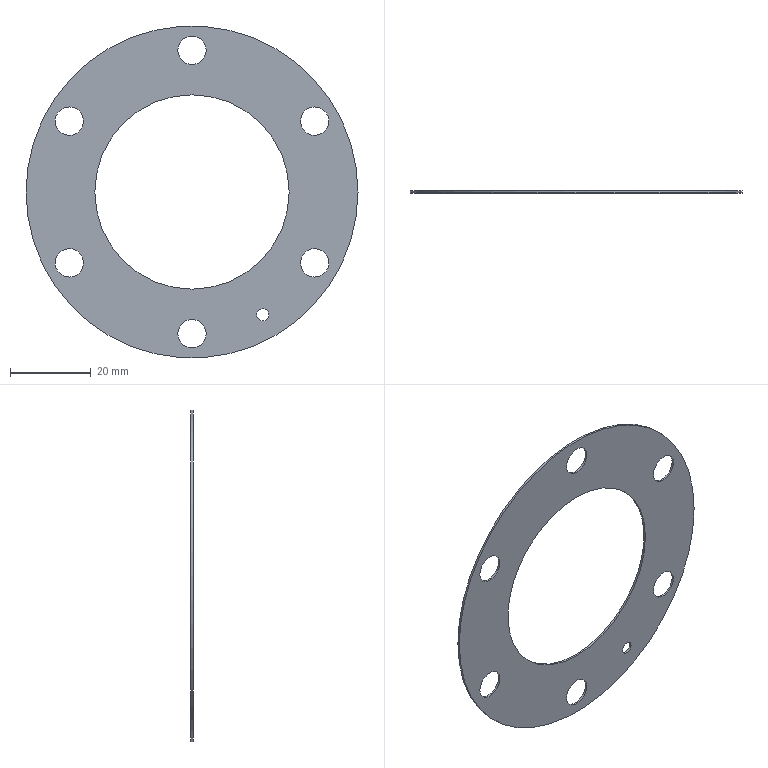Component | NX | GASKET | 1 solid | 11 faces | box 82 x 0.5 x 82 mm | volume 1617 mm3 | cylinder 9 | plane 2 | commonest cylinder face diameters 7 x6 3 x1 48 x1 82 x1
STEP:
#1=CARTESIAN_POINT('',(0.,0.,0.));
#2=DIRECTION('',(0.,0.,1.));
#3=DIRECTION('',(1.,0.,0.));
#4=AXIS2_PLACEMENT_3D('',#1,#2,#3);
#5=CARTESIAN_POINT('',(19.,-34.5,-25.811));
#6=VERTEX_POINT('',#5);
#7=CARTESIAN_POINT('',(17.5,-34.5,-25.811));
#8=DIRECTION('',(0.,1.,0.));
#9=DIRECTION('',(1.,0.,0.));
#10=AXIS2_PLACEMENT_3D('',#7,#8,#9);
#11=CIRCLE('',#10,1.5);
#12=CARTESIAN_POINT('',(17.5,-34.5,-25.811));
#13=DIRECTION('',(0.,1.,0.));
#14=DIRECTION('',(-1.,0.,0.));
#15=AXIS2_PLACEMENT_3D('',#12,#13,#14);
#16=CYLINDRICAL_SURFACE('',#15,1.5);
#17=CARTESIAN_POINT('',(3.142,0.));
#18=DIRECTION('',(1.,0.));
#19=VECTOR('',#18,1.);
#20=LINE('',#17,#19);
#21=(GEOMETRIC_REPRESENTATION_CONTEXT(2)PARAMETRIC_REPRESENTATION_CONTEXT()REPRESENTATION_CONTEXT('',''));
#22=DEFINITIONAL_REPRESENTATION('',(#20),#21);
#23=PCURVE('',#16,#22);
#24=CARTESIAN_POINT('',(15.155,-34.5,-4.25));
#25=DIRECTION('',(0.,1.,0.));
#26=DIRECTION('',(-1.,0.,0.));
#27=AXIS2_PLACEMENT_3D('',#24,#25,#26);
#28=PLANE('',#27);
#29=CARTESIAN_POINT('',(-2.345,-21.561));
#30=DIRECTION('',(-1.,0.));
#31=AXIS2_PLACEMENT_2D('',#29,#30);
#32=CIRCLE('',#31,1.5);
#33=(GEOMETRIC_REPRESENTATION_CONTEXT(2)PARAMETRIC_REPRESENTATION_CONTEXT()REPRESENTATION_CONTEXT('',''));
#34=DEFINITIONAL_REPRESENTATION('',(#32),#33);
#35=PCURVE('',#28,#34);
#36=SURFACE_CURVE('',#11,(#23,#35),.PCURVE_S1.);
#37=EDGE_CURVE('',#6,#6,#36,.T.);
#38=ORIENTED_EDGE('',*,*,#37,.T.);
#39=CARTESIAN_POINT('',(19.,-34.,-25.811));
#40=VERTEX_POINT('',#39);
#41=CARTESIAN_POINT('',(19.,-34.5,-25.811));
#42=CARTESIAN_POINT('',(19.,-34.,-25.811));
#43=B_SPLINE_CURVE_WITH_KNOTS('',1,(#41,#42),.UNSPECIFIED.,.F.,.F.,(2,2),(0.,0.5),.PIECEWISE_BEZIER_KNOTS.);
#44=CARTESIAN_POINT('',(9.425,0.));
#45=DIRECTION('',(0.,1.));
#46=VECTOR('',#45,1.);
#47=LINE('',#44,#46);
#48=(GEOMETRIC_REPRESENTATION_CONTEXT(2)PARAMETRIC_REPRESENTATION_CONTEXT()REPRESENTATION_CONTEXT('',''));
#49=DEFINITIONAL_REPRESENTATION('',(#47),#48);
#50=PCURVE('',#16,#49);
#51=CARTESIAN_POINT('',(3.142,0.));
#52=DIRECTION('',(0.,1.));
#53=VECTOR('',#52,1.);
#54=LINE('',#51,#53);
#55=(GEOMETRIC_REPRESENTATION_CONTEXT(2)PARAMETRIC_REPRESENTATION_CONTEXT()REPRESENTATION_CONTEXT('',''));
#56=DEFINITIONAL_REPRESENTATION('',(#54),#55);
#57=PCURVE('',#16,#56);
#58=SEAM_CURVE('',#43,(#50,#57),.PCURVE_S1.);
#59=EDGE_CURVE('',#6,#40,#58,.T.);
#60=ORIENTED_EDGE('',*,*,#59,.T.);
#61=CARTESIAN_POINT('',(17.5,-34.,-25.811));
#62=DIRECTION('',(0.,1.,0.));
#63=DIRECTION('',(1.,0.,0.));
#64=AXIS2_PLACEMENT_3D('',#61,#62,#63);
#65=CIRCLE('',#64,1.5);
#66=CARTESIAN_POINT('',(3.142,0.5));
#67=DIRECTION('',(1.,0.));
#68=VECTOR('',#67,1.);
#69=LINE('',#66,#68);
#70=(GEOMETRIC_REPRESENTATION_CONTEXT(2)PARAMETRIC_REPRESENTATION_CONTEXT()REPRESENTATION_CONTEXT('',''));
#71=DEFINITIONAL_REPRESENTATION('',(#69),#70);
#72=PCURVE('',#16,#71);
#73=CARTESIAN_POINT('',(15.155,-34.,-4.25));
#74=DIRECTION('',(0.,1.,0.));
#75=DIRECTION('',(-1.,0.,0.));
#76=AXIS2_PLACEMENT_3D('',#73,#74,#75);
#77=PLANE('',#76);
#78=CARTESIAN_POINT('',(-2.345,-21.561));
#79=DIRECTION('',(-1.,0.));
#80=AXIS2_PLACEMENT_2D('',#78,#79);
#81=CIRCLE('',#80,1.5);
#82=(GEOMETRIC_REPRESENTATION_CONTEXT(2)PARAMETRIC_REPRESENTATION_CONTEXT()REPRESENTATION_CONTEXT('',''));
#83=DEFINITIONAL_REPRESENTATION('',(#81),#82);
#84=PCURVE('',#77,#83);
#85=SURFACE_CURVE('',#65,(#72,#84),.PCURVE_S1.);
#86=EDGE_CURVE('',#40,#40,#85,.T.);
#87=ORIENTED_EDGE('',*,*,#86,.F.);
#88=ORIENTED_EDGE('',*,*,#59,.F.);
#89=EDGE_LOOP('',(#38,#60,#87,#88));
#90=FACE_BOUND('',#89,.F.);
#91=ADVANCED_FACE('',(#90),#16,.F.);
#92=CARTESIAN_POINT('',(-3.5,-34.5,-30.5));
#93=VERTEX_POINT('',#92);
#94=CARTESIAN_POINT('',(-0.,-34.5,-30.5));
#95=DIRECTION('',(0.,1.,0.));
#96=DIRECTION('',(-1.,0.,0.));
#97=AXIS2_PLACEMENT_3D('',#94,#95,#96);
#98=CIRCLE('',#97,3.5);
#99=CARTESIAN_POINT('',(-0.,-34.5,-30.5));
#100=DIRECTION('',(0.,1.,0.));
#101=DIRECTION('',(-1.,0.,0.));
#102=AXIS2_PLACEMENT_3D('',#99,#100,#101);
#103=CYLINDRICAL_SURFACE('',#102,3.5);
#104=CARTESIAN_POINT('',(0.,0.));
#105=DIRECTION('',(1.,0.));
#106=VECTOR('',#105,1.);
#107=LINE('',#104,#106);
#108=(GEOMETRIC_REPRESENTATION_CONTEXT(2)PARAMETRIC_REPRESENTATION_CONTEXT()REPRESENTATION_CONTEXT('',''));
#109=DEFINITIONAL_REPRESENTATION('',(#107),#108);
#110=PCURVE('',#103,#109);
#111=CARTESIAN_POINT('',(15.155,-26.25));
#112=DIRECTION('',(1.,0.));
#113=AXIS2_PLACEMENT_2D('',#111,#112);
#114=CIRCLE('',#113,3.5);
#115=(GEOMETRIC_REPRESENTATION_CONTEXT(2)PARAMETRIC_REPRESENTATION_CONTEXT()REPRESENTATION_CONTEXT('',''));
#116=DEFINITIONAL_REPRESENTATION('',(#114),#115);
#117=PCURVE('',#28,#116);
#118=SURFACE_CURVE('',#98,(#110,#117),.PCURVE_S1.);
#119=EDGE_CURVE('',#93,#93,#118,.T.);
#120=ORIENTED_EDGE('',*,*,#119,.T.);
#121=CARTESIAN_POINT('',(-3.5,-34.,-30.5));
#122=VERTEX_POINT('',#121);
#123=CARTESIAN_POINT('',(-3.5,-34.5,-30.5));
#124=CARTESIAN_POINT('',(-3.5,-34.,-30.5));
#125=B_SPLINE_CURVE_WITH_KNOTS('',1,(#123,#124),.UNSPECIFIED.,.F.,.F.,(2,2),(0.,0.5),.PIECEWISE_BEZIER_KNOTS.);
#126=CARTESIAN_POINT('',(6.283,0.));
#127=DIRECTION('',(0.,1.));
#128=VECTOR('',#127,1.);
#129=LINE('',#126,#128);
#130=(GEOMETRIC_REPRESENTATION_CONTEXT(2)PARAMETRIC_REPRESENTATION_CONTEXT()REPRESENTATION_CONTEXT('',''));
#131=DEFINITIONAL_REPRESENTATION('',(#129),#130);
#132=PCURVE('',#103,#131);
#133=CARTESIAN_POINT('',(0.,0.));
#134=DIRECTION('',(0.,1.));
#135=VECTOR('',#134,1.);
#136=LINE('',#133,#135);
#137=(GEOMETRIC_REPRESENTATION_CONTEXT(2)PARAMETRIC_REPRESENTATION_CONTEXT()REPRESENTATION_CONTEXT('',''));
#138=DEFINITIONAL_REPRESENTATION('',(#136),#137);
#139=PCURVE('',#103,#138);
#140=SEAM_CURVE('',#125,(#132,#139),.PCURVE_S1.);
#141=EDGE_CURVE('',#93,#122,#140,.T.);
#142=ORIENTED_EDGE('',*,*,#141,.T.);
#143=CARTESIAN_POINT('',(-0.,-34.,-30.5));
#144=DIRECTION('',(0.,1.,0.));
#145=DIRECTION('',(-1.,0.,0.));
#146=AXIS2_PLACEMENT_3D('',#143,#144,#145);
#147=CIRCLE('',#146,3.5);
#148=CARTESIAN_POINT('',(0.,0.5));
#149=DIRECTION('',(1.,0.));
#150=VECTOR('',#149,1.);
#151=LINE('',#148,#150);
#152=(GEOMETRIC_REPRESENTATION_CONTEXT(2)PARAMETRIC_REPRESENTATION_CONTEXT()REPRESENTATION_CONTEXT('',''));
#153=DEFINITIONAL_REPRESENTATION('',(#151),#152);
#154=PCURVE('',#103,#153);
#155=CARTESIAN_POINT('',(15.155,-26.25));
#156=DIRECTION('',(1.,0.));
#157=AXIS2_PLACEMENT_2D('',#155,#156);
#158=CIRCLE('',#157,3.5);
#159=(GEOMETRIC_REPRESENTATION_CONTEXT(2)PARAMETRIC_REPRESENTATION_CONTEXT()REPRESENTATION_CONTEXT('',''));
#160=DEFINITIONAL_REPRESENTATION('',(#158),#159);
#161=PCURVE('',#77,#160);
#162=SURFACE_CURVE('',#147,(#154,#161),.PCURVE_S1.);
#163=EDGE_CURVE('',#122,#122,#162,.T.);
#164=ORIENTED_EDGE('',*,*,#163,.F.);
#165=ORIENTED_EDGE('',*,*,#141,.F.);
#166=EDGE_LOOP('',(#120,#142,#164,#165));
#167=FACE_BOUND('',#166,.F.);
#168=ADVANCED_FACE('',(#167),#103,.F.);
#169=CARTESIAN_POINT('',(-28.561,-34.5,25.031));
#170=VERTEX_POINT('',#169);
#171=CARTESIAN_POINT('',(-30.311,-34.5,22.));
#172=DIRECTION('',(0.,1.,0.));
#173=DIRECTION('',(0.5,0.,0.866));
#174=AXIS2_PLACEMENT_3D('',#171,#172,#173);
#175=CIRCLE('',#174,3.5);
#176=CARTESIAN_POINT('',(-30.311,-34.5,22.));
#177=DIRECTION('',(0.,1.,0.));
#178=DIRECTION('',(-1.,0.,0.));
#179=AXIS2_PLACEMENT_3D('',#176,#177,#178);
#180=CYLINDRICAL_SURFACE('',#179,3.5);
#181=CARTESIAN_POINT('',(2.094,0.));
#182=DIRECTION('',(1.,0.));
#183=VECTOR('',#182,1.);
#184=LINE('',#181,#183);
#185=(GEOMETRIC_REPRESENTATION_CONTEXT(2)PARAMETRIC_REPRESENTATION_CONTEXT()REPRESENTATION_CONTEXT('',''));
#186=DEFINITIONAL_REPRESENTATION('',(#184),#185);
#187=PCURVE('',#180,#186);
#188=CARTESIAN_POINT('',(45.466,26.25));
#189=DIRECTION('',(-0.5,0.866));
#190=AXIS2_PLACEMENT_2D('',#188,#189);
#191=CIRCLE('',#190,3.5);
#192=(GEOMETRIC_REPRESENTATION_CONTEXT(2)PARAMETRIC_REPRESENTATION_CONTEXT()REPRESENTATION_CONTEXT('',''));
#193=DEFINITIONAL_REPRESENTATION('',(#191),#192);
#194=PCURVE('',#28,#193);
#195=SURFACE_CURVE('',#175,(#187,#194),.PCURVE_S1.);
#196=EDGE_CURVE('',#170,#170,#195,.T.);
#197=ORIENTED_EDGE('',*,*,#196,.T.);
#198=CARTESIAN_POINT('',(-28.561,-34.,25.031));
#199=VERTEX_POINT('',#198);
#200=CARTESIAN_POINT('',(-28.561,-34.5,25.031));
#201=CARTESIAN_POINT('',(-28.561,-34.,25.031));
#202=B_SPLINE_CURVE_WITH_KNOTS('',1,(#200,#201),.UNSPECIFIED.,.F.,.F.,(2,2),(0.,0.5),.PIECEWISE_BEZIER_KNOTS.);
#203=CARTESIAN_POINT('',(8.378,0.));
#204=DIRECTION('',(0.,1.));
#205=VECTOR('',#204,1.);
#206=LINE('',#203,#205);
#207=(GEOMETRIC_REPRESENTATION_CONTEXT(2)PARAMETRIC_REPRESENTATION_CONTEXT()REPRESENTATION_CONTEXT('',''));
#208=DEFINITIONAL_REPRESENTATION('',(#206),#207);
#209=PCURVE('',#180,#208);
#210=CARTESIAN_POINT('',(2.094,0.));
#211=DIRECTION('',(0.,1.));
#212=VECTOR('',#211,1.);
#213=LINE('',#210,#212);
#214=(GEOMETRIC_REPRESENTATION_CONTEXT(2)PARAMETRIC_REPRESENTATION_CONTEXT()REPRESENTATION_CONTEXT('',''));
#215=DEFINITIONAL_REPRESENTATION('',(#213),#214);
#216=PCURVE('',#180,#215);
#217=SEAM_CURVE('',#202,(#209,#216),.PCURVE_S1.);
#218=EDGE_CURVE('',#170,#199,#217,.T.);
#219=ORIENTED_EDGE('',*,*,#218,.T.);
#220=CARTESIAN_POINT('',(-30.311,-34.,22.));
#221=DIRECTION('',(0.,1.,0.));
#222=DIRECTION('',(0.5,0.,0.866));
#223=AXIS2_PLACEMENT_3D('',#220,#221,#222);
#224=CIRCLE('',#223,3.5);
#225=CARTESIAN_POINT('',(2.094,0.5));
#226=DIRECTION('',(1.,0.));
#227=VECTOR('',#226,1.);
#228=LINE('',#225,#227);
#229=(GEOMETRIC_REPRESENTATION_CONTEXT(2)PARAMETRIC_REPRESENTATION_CONTEXT()REPRESENTATION_CONTEXT('',''));
#230=DEFINITIONAL_REPRESENTATION('',(#228),#229);
#231=PCURVE('',#180,#230);
#232=CARTESIAN_POINT('',(45.466,26.25));
#233=DIRECTION('',(-0.5,0.866));
#234=AXIS2_PLACEMENT_2D('',#232,#233);
#235=CIRCLE('',#234,3.5);
#236=(GEOMETRIC_REPRESENTATION_CONTEXT(2)PARAMETRIC_REPRESENTATION_CONTEXT()REPRESENTATION_CONTEXT('',''));
#237=DEFINITIONAL_REPRESENTATION('',(#235),#236);
#238=PCURVE('',#77,#237);
#239=SURFACE_CURVE('',#224,(#231,#238),.PCURVE_S1.);
#240=EDGE_CURVE('',#199,#199,#239,.T.);
#241=ORIENTED_EDGE('',*,*,#240,.F.);
#242=ORIENTED_EDGE('',*,*,#218,.F.);
#243=EDGE_LOOP('',(#197,#219,#241,#242));
#244=FACE_BOUND('',#243,.F.);
#245=ADVANCED_FACE('',(#244),#180,.F.);
#246=CARTESIAN_POINT('',(-32.061,-34.5,-9.969));
#247=VERTEX_POINT('',#246);
#248=CARTESIAN_POINT('',(-30.311,-34.5,-13.));
#249=DIRECTION('',(0.,1.,0.));
#250=DIRECTION('',(-0.5,0.,0.866));
#251=AXIS2_PLACEMENT_3D('',#248,#249,#250);
#252=CIRCLE('',#251,3.5);
#253=CARTESIAN_POINT('',(-30.311,-34.5,-13.));
#254=DIRECTION('',(0.,1.,0.));
#255=DIRECTION('',(-1.,0.,0.));
#256=AXIS2_PLACEMENT_3D('',#253,#254,#255);
#257=CYLINDRICAL_SURFACE('',#256,3.5);
#258=CARTESIAN_POINT('',(1.047,0.));
#259=DIRECTION('',(1.,0.));
#260=VECTOR('',#259,1.);
#261=LINE('',#258,#260);
#262=(GEOMETRIC_REPRESENTATION_CONTEXT(2)PARAMETRIC_REPRESENTATION_CONTEXT()REPRESENTATION_CONTEXT('',''));
#263=DEFINITIONAL_REPRESENTATION('',(#261),#262);
#264=PCURVE('',#257,#263);
#265=CARTESIAN_POINT('',(45.466,-8.75));
#266=DIRECTION('',(0.5,0.866));
#267=AXIS2_PLACEMENT_2D('',#265,#266);
#268=CIRCLE('',#267,3.5);
#269=(GEOMETRIC_REPRESENTATION_CONTEXT(2)PARAMETRIC_REPRESENTATION_CONTEXT()REPRESENTATION_CONTEXT('',''));
#270=DEFINITIONAL_REPRESENTATION('',(#268),#269);
#271=PCURVE('',#28,#270);
#272=SURFACE_CURVE('',#252,(#264,#271),.PCURVE_S1.);
#273=EDGE_CURVE('',#247,#247,#272,.T.);
#274=ORIENTED_EDGE('',*,*,#273,.T.);
#275=CARTESIAN_POINT('',(-32.061,-34.,-9.969));
#276=VERTEX_POINT('',#275);
#277=CARTESIAN_POINT('',(-32.061,-34.5,-9.969));
#278=CARTESIAN_POINT('',(-32.061,-34.,-9.969));
#279=B_SPLINE_CURVE_WITH_KNOTS('',1,(#277,#278),.UNSPECIFIED.,.F.,.F.,(2,2),(0.,0.5),.PIECEWISE_BEZIER_KNOTS.);
#280=CARTESIAN_POINT('',(7.33,0.));
#281=DIRECTION('',(0.,1.));
#282=VECTOR('',#281,1.);
#283=LINE('',#280,#282);
#284=(GEOMETRIC_REPRESENTATION_CONTEXT(2)PARAMETRIC_REPRESENTATION_CONTEXT()REPRESENTATION_CONTEXT('',''));
#285=DEFINITIONAL_REPRESENTATION('',(#283),#284);
#286=PCURVE('',#257,#285);
#287=CARTESIAN_POINT('',(1.047,0.));
#288=DIRECTION('',(0.,1.));
#289=VECTOR('',#288,1.);
#290=LINE('',#287,#289);
#291=(GEOMETRIC_REPRESENTATION_CONTEXT(2)PARAMETRIC_REPRESENTATION_CONTEXT()REPRESENTATION_CONTEXT('',''));
#292=DEFINITIONAL_REPRESENTATION('',(#290),#291);
#293=PCURVE('',#257,#292);
#294=SEAM_CURVE('',#279,(#286,#293),.PCURVE_S1.);
#295=EDGE_CURVE('',#247,#276,#294,.T.);
#296=ORIENTED_EDGE('',*,*,#295,.T.);
#297=CARTESIAN_POINT('',(-30.311,-34.,-13.));
#298=DIRECTION('',(0.,1.,0.));
#299=DIRECTION('',(-0.5,0.,0.866));
#300=AXIS2_PLACEMENT_3D('',#297,#298,#299);
#301=CIRCLE('',#300,3.5);
#302=CARTESIAN_POINT('',(1.047,0.5));
#303=DIRECTION('',(1.,0.));
#304=VECTOR('',#303,1.);
#305=LINE('',#302,#304);
#306=(GEOMETRIC_REPRESENTATION_CONTEXT(2)PARAMETRIC_REPRESENTATION_CONTEXT()REPRESENTATION_CONTEXT('',''));
#307=DEFINITIONAL_REPRESENTATION('',(#305),#306);
#308=PCURVE('',#257,#307);
#309=CARTESIAN_POINT('',(45.466,-8.75));
#310=DIRECTION('',(0.5,0.866));
#311=AXIS2_PLACEMENT_2D('',#309,#310);
#312=CIRCLE('',#311,3.5);
#313=(GEOMETRIC_REPRESENTATION_CONTEXT(2)PARAMETRIC_REPRESENTATION_CONTEXT()REPRESENTATION_CONTEXT('',''));
#314=DEFINITIONAL_REPRESENTATION('',(#312),#313);
#315=PCURVE('',#77,#314);
#316=SURFACE_CURVE('',#301,(#308,#315),.PCURVE_S1.);
#317=EDGE_CURVE('',#276,#276,#316,.T.);
#318=ORIENTED_EDGE('',*,*,#317,.F.);
#319=ORIENTED_EDGE('',*,*,#295,.F.);
#320=EDGE_LOOP('',(#274,#296,#318,#319));
#321=FACE_BOUND('',#320,.F.);
#322=ADVANCED_FACE('',(#321),#257,.F.);
#323=CARTESIAN_POINT('',(24.,-34.5,4.5));
#324=VERTEX_POINT('',#323);
#325=CARTESIAN_POINT('',(-0.,-34.5,4.5));
#326=DIRECTION('',(0.,1.,0.));
#327=DIRECTION('',(1.,0.,0.));
#328=AXIS2_PLACEMENT_3D('',#325,#326,#327);
#329=CIRCLE('',#328,24.);
#330=CARTESIAN_POINT('',(-0.,-34.5,4.5));
#331=DIRECTION('',(0.,1.,0.));
#332=DIRECTION('',(-1.,0.,0.));
#333=AXIS2_PLACEMENT_3D('',#330,#331,#332);
#334=CYLINDRICAL_SURFACE('',#333,24.);
#335=CARTESIAN_POINT('',(3.142,0.));
#336=DIRECTION('',(1.,0.));
#337=VECTOR('',#336,1.);
#338=LINE('',#335,#337);
#339=(GEOMETRIC_REPRESENTATION_CONTEXT(2)PARAMETRIC_REPRESENTATION_CONTEXT()REPRESENTATION_CONTEXT('',''));
#340=DEFINITIONAL_REPRESENTATION('',(#338),#339);
#341=PCURVE('',#334,#340);
#342=CARTESIAN_POINT('',(15.155,8.75));
#343=DIRECTION('',(-1.,0.));
#344=AXIS2_PLACEMENT_2D('',#342,#343);
#345=CIRCLE('',#344,24.);
#346=(GEOMETRIC_REPRESENTATION_CONTEXT(2)PARAMETRIC_REPRESENTATION_CONTEXT()REPRESENTATION_CONTEXT('',''));
#347=DEFINITIONAL_REPRESENTATION('',(#345),#346);
#348=PCURVE('',#28,#347);
#349=SURFACE_CURVE('',#329,(#341,#348),.PCURVE_S1.);
#350=EDGE_CURVE('',#324,#324,#349,.T.);
#351=ORIENTED_EDGE('',*,*,#350,.T.);
#352=CARTESIAN_POINT('',(24.,-34.,4.5));
#353=VERTEX_POINT('',#352);
#354=CARTESIAN_POINT('',(24.,-34.5,4.5));
#355=CARTESIAN_POINT('',(24.,-34.,4.5));
#356=B_SPLINE_CURVE_WITH_KNOTS('',1,(#354,#355),.UNSPECIFIED.,.F.,.F.,(2,2),(0.,0.5),.PIECEWISE_BEZIER_KNOTS.);
#357=CARTESIAN_POINT('',(9.425,0.));
#358=DIRECTION('',(0.,1.));
#359=VECTOR('',#358,1.);
#360=LINE('',#357,#359);
#361=(GEOMETRIC_REPRESENTATION_CONTEXT(2)PARAMETRIC_REPRESENTATION_CONTEXT()REPRESENTATION_CONTEXT('',''));
#362=DEFINITIONAL_REPRESENTATION('',(#360),#361);
#363=PCURVE('',#334,#362);
#364=CARTESIAN_POINT('',(3.142,0.));
#365=DIRECTION('',(0.,1.));
#366=VECTOR('',#365,1.);
#367=LINE('',#364,#366);
#368=(GEOMETRIC_REPRESENTATION_CONTEXT(2)PARAMETRIC_REPRESENTATION_CONTEXT()REPRESENTATION_CONTEXT('',''));
#369=DEFINITIONAL_REPRESENTATION('',(#367),#368);
#370=PCURVE('',#334,#369);
#371=SEAM_CURVE('',#356,(#363,#370),.PCURVE_S1.);
#372=EDGE_CURVE('',#324,#353,#371,.T.);
#373=ORIENTED_EDGE('',*,*,#372,.T.);
#374=CARTESIAN_POINT('',(-0.,-34.,4.5));
#375=DIRECTION('',(0.,1.,0.));
#376=DIRECTION('',(1.,0.,0.));
#377=AXIS2_PLACEMENT_3D('',#374,#375,#376);
#378=CIRCLE('',#377,24.);
#379=CARTESIAN_POINT('',(3.142,0.5));
#380=DIRECTION('',(1.,0.));
#381=VECTOR('',#380,1.);
#382=LINE('',#379,#381);
#383=(GEOMETRIC_REPRESENTATION_CONTEXT(2)PARAMETRIC_REPRESENTATION_CONTEXT()REPRESENTATION_CONTEXT('',''));
#384=DEFINITIONAL_REPRESENTATION('',(#382),#383);
#385=PCURVE('',#334,#384);
#386=CARTESIAN_POINT('',(15.155,8.75));
#387=DIRECTION('',(-1.,0.));
#388=AXIS2_PLACEMENT_2D('',#386,#387);
#389=CIRCLE('',#388,24.);
#390=(GEOMETRIC_REPRESENTATION_CONTEXT(2)PARAMETRIC_REPRESENTATION_CONTEXT()REPRESENTATION_CONTEXT('',''));
#391=DEFINITIONAL_REPRESENTATION('',(#389),#390);
#392=PCURVE('',#77,#391);
#393=SURFACE_CURVE('',#378,(#385,#392),.PCURVE_S1.);
#394=EDGE_CURVE('',#353,#353,#393,.T.);
#395=ORIENTED_EDGE('',*,*,#394,.F.);
#396=ORIENTED_EDGE('',*,*,#372,.F.);
#397=EDGE_LOOP('',(#351,#373,#395,#396));
#398=FACE_BOUND('',#397,.F.);
#399=ADVANCED_FACE('',(#398),#334,.F.);
#400=CARTESIAN_POINT('',(3.5,-34.5,39.5));
#401=VERTEX_POINT('',#400);
#402=CARTESIAN_POINT('',(-0.,-34.5,39.5));
#403=DIRECTION('',(0.,1.,0.));
#404=DIRECTION('',(1.,0.,0.));
#405=AXIS2_PLACEMENT_3D('',#402,#403,#404);
#406=CIRCLE('',#405,3.5);
#407=CARTESIAN_POINT('',(-0.,-34.5,39.5));
#408=DIRECTION('',(0.,1.,0.));
#409=DIRECTION('',(-1.,0.,0.));
#410=AXIS2_PLACEMENT_3D('',#407,#408,#409);
#411=CYLINDRICAL_SURFACE('',#410,3.5);
#412=CARTESIAN_POINT('',(3.142,0.));
#413=DIRECTION('',(1.,0.));
#414=VECTOR('',#413,1.);
#415=LINE('',#412,#414);
#416=(GEOMETRIC_REPRESENTATION_CONTEXT(2)PARAMETRIC_REPRESENTATION_CONTEXT()REPRESENTATION_CONTEXT('',''));
#417=DEFINITIONAL_REPRESENTATION('',(#415),#416);
#418=PCURVE('',#411,#417);
#419=CARTESIAN_POINT('',(15.155,43.75));
#420=DIRECTION('',(-1.,0.));
#421=AXIS2_PLACEMENT_2D('',#419,#420);
#422=CIRCLE('',#421,3.5);
#423=(GEOMETRIC_REPRESENTATION_CONTEXT(2)PARAMETRIC_REPRESENTATION_CONTEXT()REPRESENTATION_CONTEXT('',''));
#424=DEFINITIONAL_REPRESENTATION('',(#422),#423);
#425=PCURVE('',#28,#424);
#426=SURFACE_CURVE('',#406,(#418,#425),.PCURVE_S1.);
#427=EDGE_CURVE('',#401,#401,#426,.T.);
#428=ORIENTED_EDGE('',*,*,#427,.T.);
#429=CARTESIAN_POINT('',(3.5,-34.,39.5));
#430=VERTEX_POINT('',#429);
#431=CARTESIAN_POINT('',(3.5,-34.5,39.5));
#432=CARTESIAN_POINT('',(3.5,-34.,39.5));
#433=B_SPLINE_CURVE_WITH_KNOTS('',1,(#431,#432),.UNSPECIFIED.,.F.,.F.,(2,2),(0.,0.5),.PIECEWISE_BEZIER_KNOTS.);
#434=CARTESIAN_POINT('',(9.425,0.));
#435=DIRECTION('',(0.,1.));
#436=VECTOR('',#435,1.);
#437=LINE('',#434,#436);
#438=(GEOMETRIC_REPRESENTATION_CONTEXT(2)PARAMETRIC_REPRESENTATION_CONTEXT()REPRESENTATION_CONTEXT('',''));
#439=DEFINITIONAL_REPRESENTATION('',(#437),#438);
#440=PCURVE('',#411,#439);
#441=CARTESIAN_POINT('',(3.142,0.));
#442=DIRECTION('',(0.,1.));
#443=VECTOR('',#442,1.);
#444=LINE('',#441,#443);
#445=(GEOMETRIC_REPRESENTATION_CONTEXT(2)PARAMETRIC_REPRESENTATION_CONTEXT()REPRESENTATION_CONTEXT('',''));
#446=DEFINITIONAL_REPRESENTATION('',(#444),#445);
#447=PCURVE('',#411,#446);
#448=SEAM_CURVE('',#433,(#440,#447),.PCURVE_S1.);
#449=EDGE_CURVE('',#401,#430,#448,.T.);
#450=ORIENTED_EDGE('',*,*,#449,.T.);
#451=CARTESIAN_POINT('',(-0.,-34.,39.5));
#452=DIRECTION('',(0.,1.,0.));
#453=DIRECTION('',(1.,0.,0.));
#454=AXIS2_PLACEMENT_3D('',#451,#452,#453);
#455=CIRCLE('',#454,3.5);
#456=CARTESIAN_POINT('',(3.142,0.5));
#457=DIRECTION('',(1.,0.));
#458=VECTOR('',#457,1.);
#459=LINE('',#456,#458);
#460=(GEOMETRIC_REPRESENTATION_CONTEXT(2)PARAMETRIC_REPRESENTATION_CONTEXT()REPRESENTATION_CONTEXT('',''));
#461=DEFINITIONAL_REPRESENTATION('',(#459),#460);
#462=PCURVE('',#411,#461);
#463=CARTESIAN_POINT('',(15.155,43.75));
#464=DIRECTION('',(-1.,0.));
#465=AXIS2_PLACEMENT_2D('',#463,#464);
#466=CIRCLE('',#465,3.5);
#467=(GEOMETRIC_REPRESENTATION_CONTEXT(2)PARAMETRIC_REPRESENTATION_CONTEXT()REPRESENTATION_CONTEXT('',''));
#468=DEFINITIONAL_REPRESENTATION('',(#466),#467);
#469=PCURVE('',#77,#468);
#470=SURFACE_CURVE('',#455,(#462,#469),.PCURVE_S1.);
#471=EDGE_CURVE('',#430,#430,#470,.T.);
#472=ORIENTED_EDGE('',*,*,#471,.F.);
#473=ORIENTED_EDGE('',*,*,#449,.F.);
#474=EDGE_LOOP('',(#428,#450,#472,#473));
#475=FACE_BOUND('',#474,.F.);
#476=ADVANCED_FACE('',(#475),#411,.F.);
#477=CARTESIAN_POINT('',(28.561,-34.5,-16.031));
#478=VERTEX_POINT('',#477);
#479=CARTESIAN_POINT('',(30.311,-34.5,-13.));
#480=DIRECTION('',(0.,1.,0.));
#481=DIRECTION('',(-0.5,0.,-0.866));
#482=AXIS2_PLACEMENT_3D('',#479,#480,#481);
#483=CIRCLE('',#482,3.5);
#484=CARTESIAN_POINT('',(30.311,-34.5,-13.));
#485=DIRECTION('',(0.,1.,0.));
#486=DIRECTION('',(-1.,0.,0.));
#487=AXIS2_PLACEMENT_3D('',#484,#485,#486);
#488=CYLINDRICAL_SURFACE('',#487,3.5);
#489=CARTESIAN_POINT('',(5.236,0.));
#490=DIRECTION('',(1.,0.));
#491=VECTOR('',#490,1.);
#492=LINE('',#489,#491);
#493=(GEOMETRIC_REPRESENTATION_CONTEXT(2)PARAMETRIC_REPRESENTATION_CONTEXT()REPRESENTATION_CONTEXT('',''));
#494=DEFINITIONAL_REPRESENTATION('',(#492),#493);
#495=PCURVE('',#488,#494);
#496=CARTESIAN_POINT('',(-15.155,-8.75));
#497=DIRECTION('',(0.5,-0.866));
#498=AXIS2_PLACEMENT_2D('',#496,#497);
#499=CIRCLE('',#498,3.5);
#500=(GEOMETRIC_REPRESENTATION_CONTEXT(2)PARAMETRIC_REPRESENTATION_CONTEXT()REPRESENTATION_CONTEXT('',''));
#501=DEFINITIONAL_REPRESENTATION('',(#499),#500);
#502=PCURVE('',#28,#501);
#503=SURFACE_CURVE('',#483,(#495,#502),.PCURVE_S1.);
#504=EDGE_CURVE('',#478,#478,#503,.T.);
#505=ORIENTED_EDGE('',*,*,#504,.T.);
#506=CARTESIAN_POINT('',(28.561,-34.,-16.031));
#507=VERTEX_POINT('',#506);
#508=CARTESIAN_POINT('',(28.561,-34.5,-16.031));
#509=CARTESIAN_POINT('',(28.561,-34.,-16.031));
#510=B_SPLINE_CURVE_WITH_KNOTS('',1,(#508,#509),.UNSPECIFIED.,.F.,.F.,(2,2),(0.,0.5),.PIECEWISE_BEZIER_KNOTS.);
#511=CARTESIAN_POINT('',(11.519,0.));
#512=DIRECTION('',(0.,1.));
#513=VECTOR('',#512,1.);
#514=LINE('',#511,#513);
#515=(GEOMETRIC_REPRESENTATION_CONTEXT(2)PARAMETRIC_REPRESENTATION_CONTEXT()REPRESENTATION_CONTEXT('',''));
#516=DEFINITIONAL_REPRESENTATION('',(#514),#515);
#517=PCURVE('',#488,#516);
#518=CARTESIAN_POINT('',(5.236,0.));
#519=DIRECTION('',(0.,1.));
#520=VECTOR('',#519,1.);
#521=LINE('',#518,#520);
#522=(GEOMETRIC_REPRESENTATION_CONTEXT(2)PARAMETRIC_REPRESENTATION_CONTEXT()REPRESENTATION_CONTEXT('',''));
#523=DEFINITIONAL_REPRESENTATION('',(#521),#522);
#524=PCURVE('',#488,#523);
#525=SEAM_CURVE('',#510,(#517,#524),.PCURVE_S1.);
#526=EDGE_CURVE('',#478,#507,#525,.T.);
#527=ORIENTED_EDGE('',*,*,#526,.T.);
#528=CARTESIAN_POINT('',(30.311,-34.,-13.));
#529=DIRECTION('',(0.,1.,0.));
#530=DIRECTION('',(-0.5,0.,-0.866));
#531=AXIS2_PLACEMENT_3D('',#528,#529,#530);
#532=CIRCLE('',#531,3.5);
#533=CARTESIAN_POINT('',(5.236,0.5));
#534=DIRECTION('',(1.,0.));
#535=VECTOR('',#534,1.);
#536=LINE('',#533,#535);
#537=(GEOMETRIC_REPRESENTATION_CONTEXT(2)PARAMETRIC_REPRESENTATION_CONTEXT()REPRESENTATION_CONTEXT('',''));
#538=DEFINITIONAL_REPRESENTATION('',(#536),#537);
#539=PCURVE('',#488,#538);
#540=CARTESIAN_POINT('',(-15.155,-8.75));
#541=DIRECTION('',(0.5,-0.866));
#542=AXIS2_PLACEMENT_2D('',#540,#541);
#543=CIRCLE('',#542,3.5);
#544=(GEOMETRIC_REPRESENTATION_CONTEXT(2)PARAMETRIC_REPRESENTATION_CONTEXT()REPRESENTATION_CONTEXT('',''));
#545=DEFINITIONAL_REPRESENTATION('',(#543),#544);
#546=PCURVE('',#77,#545);
#547=SURFACE_CURVE('',#532,(#539,#546),.PCURVE_S1.);
#548=EDGE_CURVE('',#507,#507,#547,.T.);
#549=ORIENTED_EDGE('',*,*,#548,.F.);
#550=ORIENTED_EDGE('',*,*,#526,.F.);
#551=EDGE_LOOP('',(#505,#527,#549,#550));
#552=FACE_BOUND('',#551,.F.);
#553=ADVANCED_FACE('',(#552),#488,.F.);
#554=CARTESIAN_POINT('',(41.,-34.5,4.5));
#555=VERTEX_POINT('',#554);
#556=CARTESIAN_POINT('',(-0.,-34.5,4.5));
#557=DIRECTION('',(0.,1.,0.));
#558=DIRECTION('',(1.,0.,0.));
#559=AXIS2_PLACEMENT_3D('',#556,#557,#558);
#560=CIRCLE('',#559,41.);
#561=CARTESIAN_POINT('',(-0.,-34.5,4.5));
#562=DIRECTION('',(0.,1.,0.));
#563=DIRECTION('',(-1.,0.,0.));
#564=AXIS2_PLACEMENT_3D('',#561,#562,#563);
#565=CYLINDRICAL_SURFACE('',#564,41.);
#566=CARTESIAN_POINT('',(3.142,0.));
#567=DIRECTION('',(1.,0.));
#568=VECTOR('',#567,1.);
#569=LINE('',#566,#568);
#570=(GEOMETRIC_REPRESENTATION_CONTEXT(2)PARAMETRIC_REPRESENTATION_CONTEXT()REPRESENTATION_CONTEXT('',''));
#571=DEFINITIONAL_REPRESENTATION('',(#569),#570);
#572=PCURVE('',#565,#571);
#573=CARTESIAN_POINT('',(15.155,8.75));
#574=DIRECTION('',(-1.,0.));
#575=AXIS2_PLACEMENT_2D('',#573,#574);
#576=CIRCLE('',#575,41.);
#577=(GEOMETRIC_REPRESENTATION_CONTEXT(2)PARAMETRIC_REPRESENTATION_CONTEXT()REPRESENTATION_CONTEXT('',''));
#578=DEFINITIONAL_REPRESENTATION('',(#576),#577);
#579=PCURVE('',#28,#578);
#580=SURFACE_CURVE('',#560,(#572,#579),.PCURVE_S1.);
#581=EDGE_CURVE('',#555,#555,#580,.T.);
#582=ORIENTED_EDGE('',*,*,#581,.T.);
#583=CARTESIAN_POINT('',(41.,-34.,4.5));
#584=VERTEX_POINT('',#583);
#585=CARTESIAN_POINT('',(41.,-34.5,4.5));
#586=CARTESIAN_POINT('',(41.,-34.,4.5));
#587=B_SPLINE_CURVE_WITH_KNOTS('',1,(#585,#586),.UNSPECIFIED.,.F.,.F.,(2,2),(0.,0.5),.PIECEWISE_BEZIER_KNOTS.);
#588=CARTESIAN_POINT('',(9.425,0.));
#589=DIRECTION('',(0.,1.));
#590=VECTOR('',#589,1.);
#591=LINE('',#588,#590);
#592=(GEOMETRIC_REPRESENTATION_CONTEXT(2)PARAMETRIC_REPRESENTATION_CONTEXT()REPRESENTATION_CONTEXT('',''));
#593=DEFINITIONAL_REPRESENTATION('',(#591),#592);
#594=PCURVE('',#565,#593);
#595=CARTESIAN_POINT('',(3.142,0.));
#596=DIRECTION('',(0.,1.));
#597=VECTOR('',#596,1.);
#598=LINE('',#595,#597);
#599=(GEOMETRIC_REPRESENTATION_CONTEXT(2)PARAMETRIC_REPRESENTATION_CONTEXT()REPRESENTATION_CONTEXT('',''));
#600=DEFINITIONAL_REPRESENTATION('',(#598),#599);
#601=PCURVE('',#565,#600);
#602=SEAM_CURVE('',#587,(#594,#601),.PCURVE_S1.);
#603=EDGE_CURVE('',#555,#584,#602,.T.);
#604=ORIENTED_EDGE('',*,*,#603,.T.);
#605=CARTESIAN_POINT('',(-0.,-34.,4.5));
#606=DIRECTION('',(0.,1.,0.));
#607=DIRECTION('',(1.,0.,0.));
#608=AXIS2_PLACEMENT_3D('',#605,#606,#607);
#609=CIRCLE('',#608,41.);
#610=CARTESIAN_POINT('',(3.142,0.5));
#611=DIRECTION('',(1.,0.));
#612=VECTOR('',#611,1.);
#613=LINE('',#610,#612);
#614=(GEOMETRIC_REPRESENTATION_CONTEXT(2)PARAMETRIC_REPRESENTATION_CONTEXT()REPRESENTATION_CONTEXT('',''));
#615=DEFINITIONAL_REPRESENTATION('',(#613),#614);
#616=PCURVE('',#565,#615);
#617=CARTESIAN_POINT('',(15.155,8.75));
#618=DIRECTION('',(-1.,0.));
#619=AXIS2_PLACEMENT_2D('',#617,#618);
#620=CIRCLE('',#619,41.);
#621=(GEOMETRIC_REPRESENTATION_CONTEXT(2)PARAMETRIC_REPRESENTATION_CONTEXT()REPRESENTATION_CONTEXT('',''));
#622=DEFINITIONAL_REPRESENTATION('',(#620),#621);
#623=PCURVE('',#77,#622);
#624=SURFACE_CURVE('',#609,(#616,#623),.PCURVE_S1.);
#625=EDGE_CURVE('',#584,#584,#624,.T.);
#626=ORIENTED_EDGE('',*,*,#625,.F.);
#627=ORIENTED_EDGE('',*,*,#603,.F.);
#628=EDGE_LOOP('',(#582,#604,#626,#627));
#629=FACE_BOUND('',#628,.T.);
#630=ADVANCED_FACE('',(#629),#565,.T.);
#631=CARTESIAN_POINT('',(32.061,-34.5,18.969));
#632=VERTEX_POINT('',#631);
#633=CARTESIAN_POINT('',(30.311,-34.5,22.));
#634=DIRECTION('',(0.,1.,0.));
#635=DIRECTION('',(0.5,0.,-0.866));
#636=AXIS2_PLACEMENT_3D('',#633,#634,#635);
#637=CIRCLE('',#636,3.5);
#638=CARTESIAN_POINT('',(30.311,-34.5,22.));
#639=DIRECTION('',(0.,1.,0.));
#640=DIRECTION('',(-1.,0.,0.));
#641=AXIS2_PLACEMENT_3D('',#638,#639,#640);
#642=CYLINDRICAL_SURFACE('',#641,3.5);
#643=CARTESIAN_POINT('',(4.189,0.));
#644=DIRECTION('',(1.,0.));
#645=VECTOR('',#644,1.);
#646=LINE('',#643,#645);
#647=(GEOMETRIC_REPRESENTATION_CONTEXT(2)PARAMETRIC_REPRESENTATION_CONTEXT()REPRESENTATION_CONTEXT('',''));
#648=DEFINITIONAL_REPRESENTATION('',(#646),#647);
#649=PCURVE('',#642,#648);
#650=CARTESIAN_POINT('',(-15.155,26.25));
#651=DIRECTION('',(-0.5,-0.866));
#652=AXIS2_PLACEMENT_2D('',#650,#651);
#653=CIRCLE('',#652,3.5);
#654=(GEOMETRIC_REPRESENTATION_CONTEXT(2)PARAMETRIC_REPRESENTATION_CONTEXT()REPRESENTATION_CONTEXT('',''));
#655=DEFINITIONAL_REPRESENTATION('',(#653),#654);
#656=PCURVE('',#28,#655);
#657=SURFACE_CURVE('',#637,(#649,#656),.PCURVE_S1.);
#658=EDGE_CURVE('',#632,#632,#657,.T.);
#659=ORIENTED_EDGE('',*,*,#658,.T.);
#660=CARTESIAN_POINT('',(32.061,-34.,18.969));
#661=VERTEX_POINT('',#660);
#662=CARTESIAN_POINT('',(32.061,-34.5,18.969));
#663=CARTESIAN_POINT('',(32.061,-34.,18.969));
#664=B_SPLINE_CURVE_WITH_KNOTS('',1,(#662,#663),.UNSPECIFIED.,.F.,.F.,(2,2),(0.,0.5),.PIECEWISE_BEZIER_KNOTS.);
#665=CARTESIAN_POINT('',(10.472,0.));
#666=DIRECTION('',(0.,1.));
#667=VECTOR('',#666,1.);
#668=LINE('',#665,#667);
#669=(GEOMETRIC_REPRESENTATION_CONTEXT(2)PARAMETRIC_REPRESENTATION_CONTEXT()REPRESENTATION_CONTEXT('',''));
#670=DEFINITIONAL_REPRESENTATION('',(#668),#669);
#671=PCURVE('',#642,#670);
#672=CARTESIAN_POINT('',(4.189,0.));
#673=DIRECTION('',(0.,1.));
#674=VECTOR('',#673,1.);
#675=LINE('',#672,#674);
#676=(GEOMETRIC_REPRESENTATION_CONTEXT(2)PARAMETRIC_REPRESENTATION_CONTEXT()REPRESENTATION_CONTEXT('',''));
#677=DEFINITIONAL_REPRESENTATION('',(#675),#676);
#678=PCURVE('',#642,#677);
#679=SEAM_CURVE('',#664,(#671,#678),.PCURVE_S1.);
#680=EDGE_CURVE('',#632,#661,#679,.T.);
#681=ORIENTED_EDGE('',*,*,#680,.T.);
#682=CARTESIAN_POINT('',(30.311,-34.,22.));
#683=DIRECTION('',(0.,1.,0.));
#684=DIRECTION('',(0.5,0.,-0.866));
#685=AXIS2_PLACEMENT_3D('',#682,#683,#684);
#686=CIRCLE('',#685,3.5);
#687=CARTESIAN_POINT('',(4.189,0.5));
#688=DIRECTION('',(1.,0.));
#689=VECTOR('',#688,1.);
#690=LINE('',#687,#689);
#691=(GEOMETRIC_REPRESENTATION_CONTEXT(2)PARAMETRIC_REPRESENTATION_CONTEXT()REPRESENTATION_CONTEXT('',''));
#692=DEFINITIONAL_REPRESENTATION('',(#690),#691);
#693=PCURVE('',#642,#692);
#694=CARTESIAN_POINT('',(-15.155,26.25));
#695=DIRECTION('',(-0.5,-0.866));
#696=AXIS2_PLACEMENT_2D('',#694,#695);
#697=CIRCLE('',#696,3.5);
#698=(GEOMETRIC_REPRESENTATION_CONTEXT(2)PARAMETRIC_REPRESENTATION_CONTEXT()REPRESENTATION_CONTEXT('',''));
#699=DEFINITIONAL_REPRESENTATION('',(#697),#698);
#700=PCURVE('',#77,#699);
#701=SURFACE_CURVE('',#686,(#693,#700),.PCURVE_S1.);
#702=EDGE_CURVE('',#661,#661,#701,.T.);
#703=ORIENTED_EDGE('',*,*,#702,.F.);
#704=ORIENTED_EDGE('',*,*,#680,.F.);
#705=EDGE_LOOP('',(#659,#681,#703,#704));
#706=FACE_BOUND('',#705,.F.);
#707=ADVANCED_FACE('',(#706),#642,.F.);
#708=ORIENTED_EDGE('',*,*,#581,.F.);
#709=EDGE_LOOP('',(#708));
#710=FACE_BOUND('',#709,.T.);
#711=ORIENTED_EDGE('',*,*,#504,.T.);
#712=EDGE_LOOP('',(#711));
#713=FACE_BOUND('',#712,.T.);
#714=ORIENTED_EDGE('',*,*,#427,.T.);
#715=EDGE_LOOP('',(#714));
#716=FACE_BOUND('',#715,.T.);
#717=ORIENTED_EDGE('',*,*,#350,.T.);
#718=EDGE_LOOP('',(#717));
#719=FACE_BOUND('',#718,.T.);
#720=ORIENTED_EDGE('',*,*,#273,.T.);
#721=EDGE_LOOP('',(#720));
#722=FACE_BOUND('',#721,.T.);
#723=ORIENTED_EDGE('',*,*,#196,.T.);
#724=EDGE_LOOP('',(#723));
#725=FACE_BOUND('',#724,.T.);
#726=ORIENTED_EDGE('',*,*,#119,.T.);
#727=EDGE_LOOP('',(#726));
#728=FACE_BOUND('',#727,.T.);
#729=ORIENTED_EDGE('',*,*,#37,.T.);
#730=EDGE_LOOP('',(#729));
#731=FACE_BOUND('',#730,.T.);
#732=ORIENTED_EDGE('',*,*,#658,.T.);
#733=EDGE_LOOP('',(#732));
#734=FACE_BOUND('',#733,.T.);
#735=ADVANCED_FACE('',(#710,#713,#716,#719,#722,#725,#728,#731,#734),#28,.F.);
#736=ORIENTED_EDGE('',*,*,#625,.T.);
#737=EDGE_LOOP('',(#736));
#738=FACE_BOUND('',#737,.T.);
#739=ORIENTED_EDGE('',*,*,#548,.F.);
#740=EDGE_LOOP('',(#739));
#741=FACE_BOUND('',#740,.T.);
#742=ORIENTED_EDGE('',*,*,#471,.F.);
#743=EDGE_LOOP('',(#742));
#744=FACE_BOUND('',#743,.T.);
#745=ORIENTED_EDGE('',*,*,#394,.F.);
#746=EDGE_LOOP('',(#745));
#747=FACE_BOUND('',#746,.T.);
#748=ORIENTED_EDGE('',*,*,#317,.F.);
#749=EDGE_LOOP('',(#748));
#750=FACE_BOUND('',#749,.T.);
#751=ORIENTED_EDGE('',*,*,#240,.F.);
#752=EDGE_LOOP('',(#751));
#753=FACE_BOUND('',#752,.T.);
#754=ORIENTED_EDGE('',*,*,#163,.F.);
#755=EDGE_LOOP('',(#754));
#756=FACE_BOUND('',#755,.T.);
#757=ORIENTED_EDGE('',*,*,#86,.F.);
#758=EDGE_LOOP('',(#757));
#759=FACE_BOUND('',#758,.T.);
#760=ORIENTED_EDGE('',*,*,#702,.F.);
#761=EDGE_LOOP('',(#760));
#762=FACE_BOUND('',#761,.T.);
#763=ADVANCED_FACE('',(#738,#741,#744,#747,#750,#753,#756,#759,#762),#77,.T.);
#764=CLOSED_SHELL('',(#91,#168,#245,#322,#399,#476,#553,#630,#707,#735,#763));
#765=MANIFOLD_SOLID_BREP('',#764);
#766=(LENGTH_UNIT()NAMED_UNIT(*)SI_UNIT(.MILLI.,.METRE.));
#767=UNCERTAINTY_MEASURE_WITH_UNIT(LENGTH_MEASURE(0.00001),#766,'','');
#768=(NAMED_UNIT(*)PLANE_ANGLE_UNIT()SI_UNIT($,.RADIAN.));
#769=(NAMED_UNIT(*)SI_UNIT($,.STERADIAN.)SOLID_ANGLE_UNIT());
#770=(GEOMETRIC_REPRESENTATION_CONTEXT(3)GLOBAL_UNCERTAINTY_ASSIGNED_CONTEXT((#767))GLOBAL_UNIT_ASSIGNED_CONTEXT((#766,#768,#769))REPRESENTATION_CONTEXT('',''));
#771=ADVANCED_BREP_SHAPE_REPRESENTATION('',(#4,#765),#770);